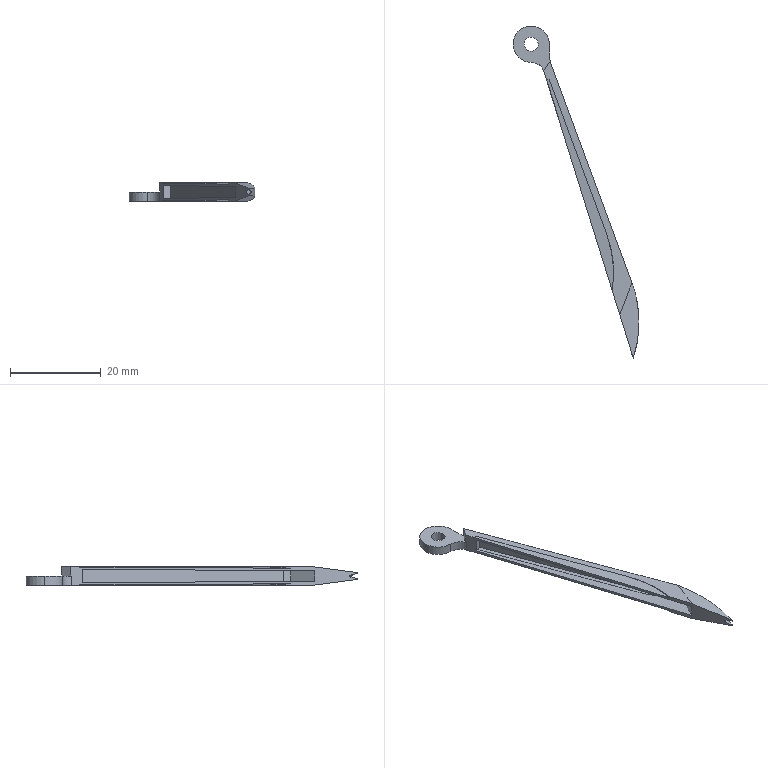Component | NX | 03 | 1 solid | 34 faces | volume 484 mm3 | plane 23 | cylinder 11 | commonest cylinder face diameters 8 x3 50 x3 6 x2 49 x1 1 x1 3.1 x1